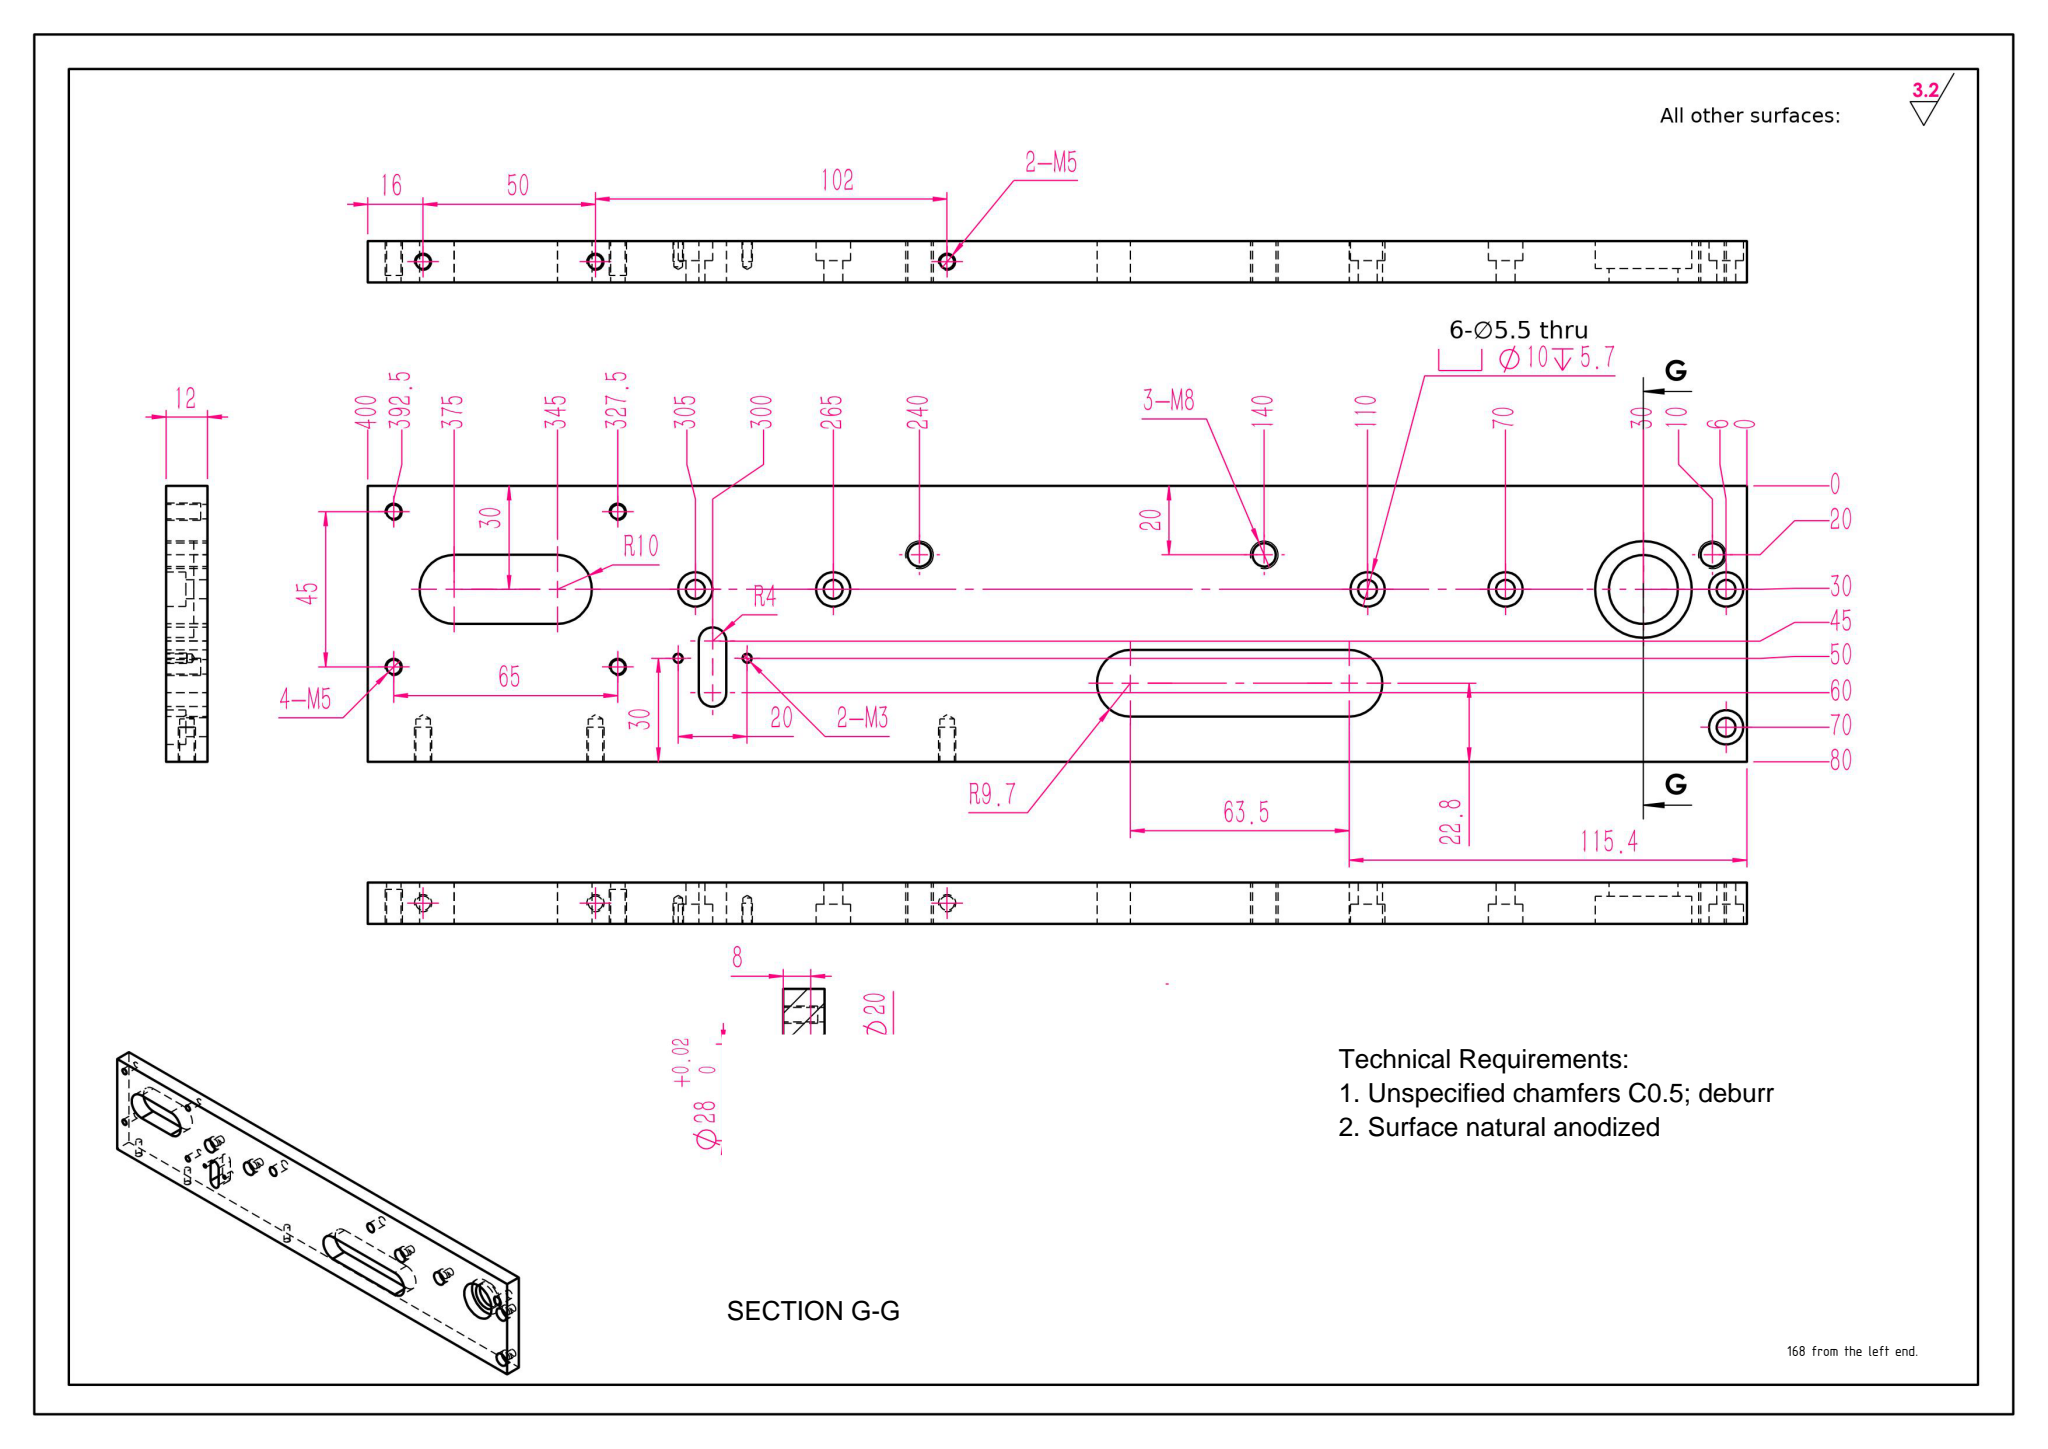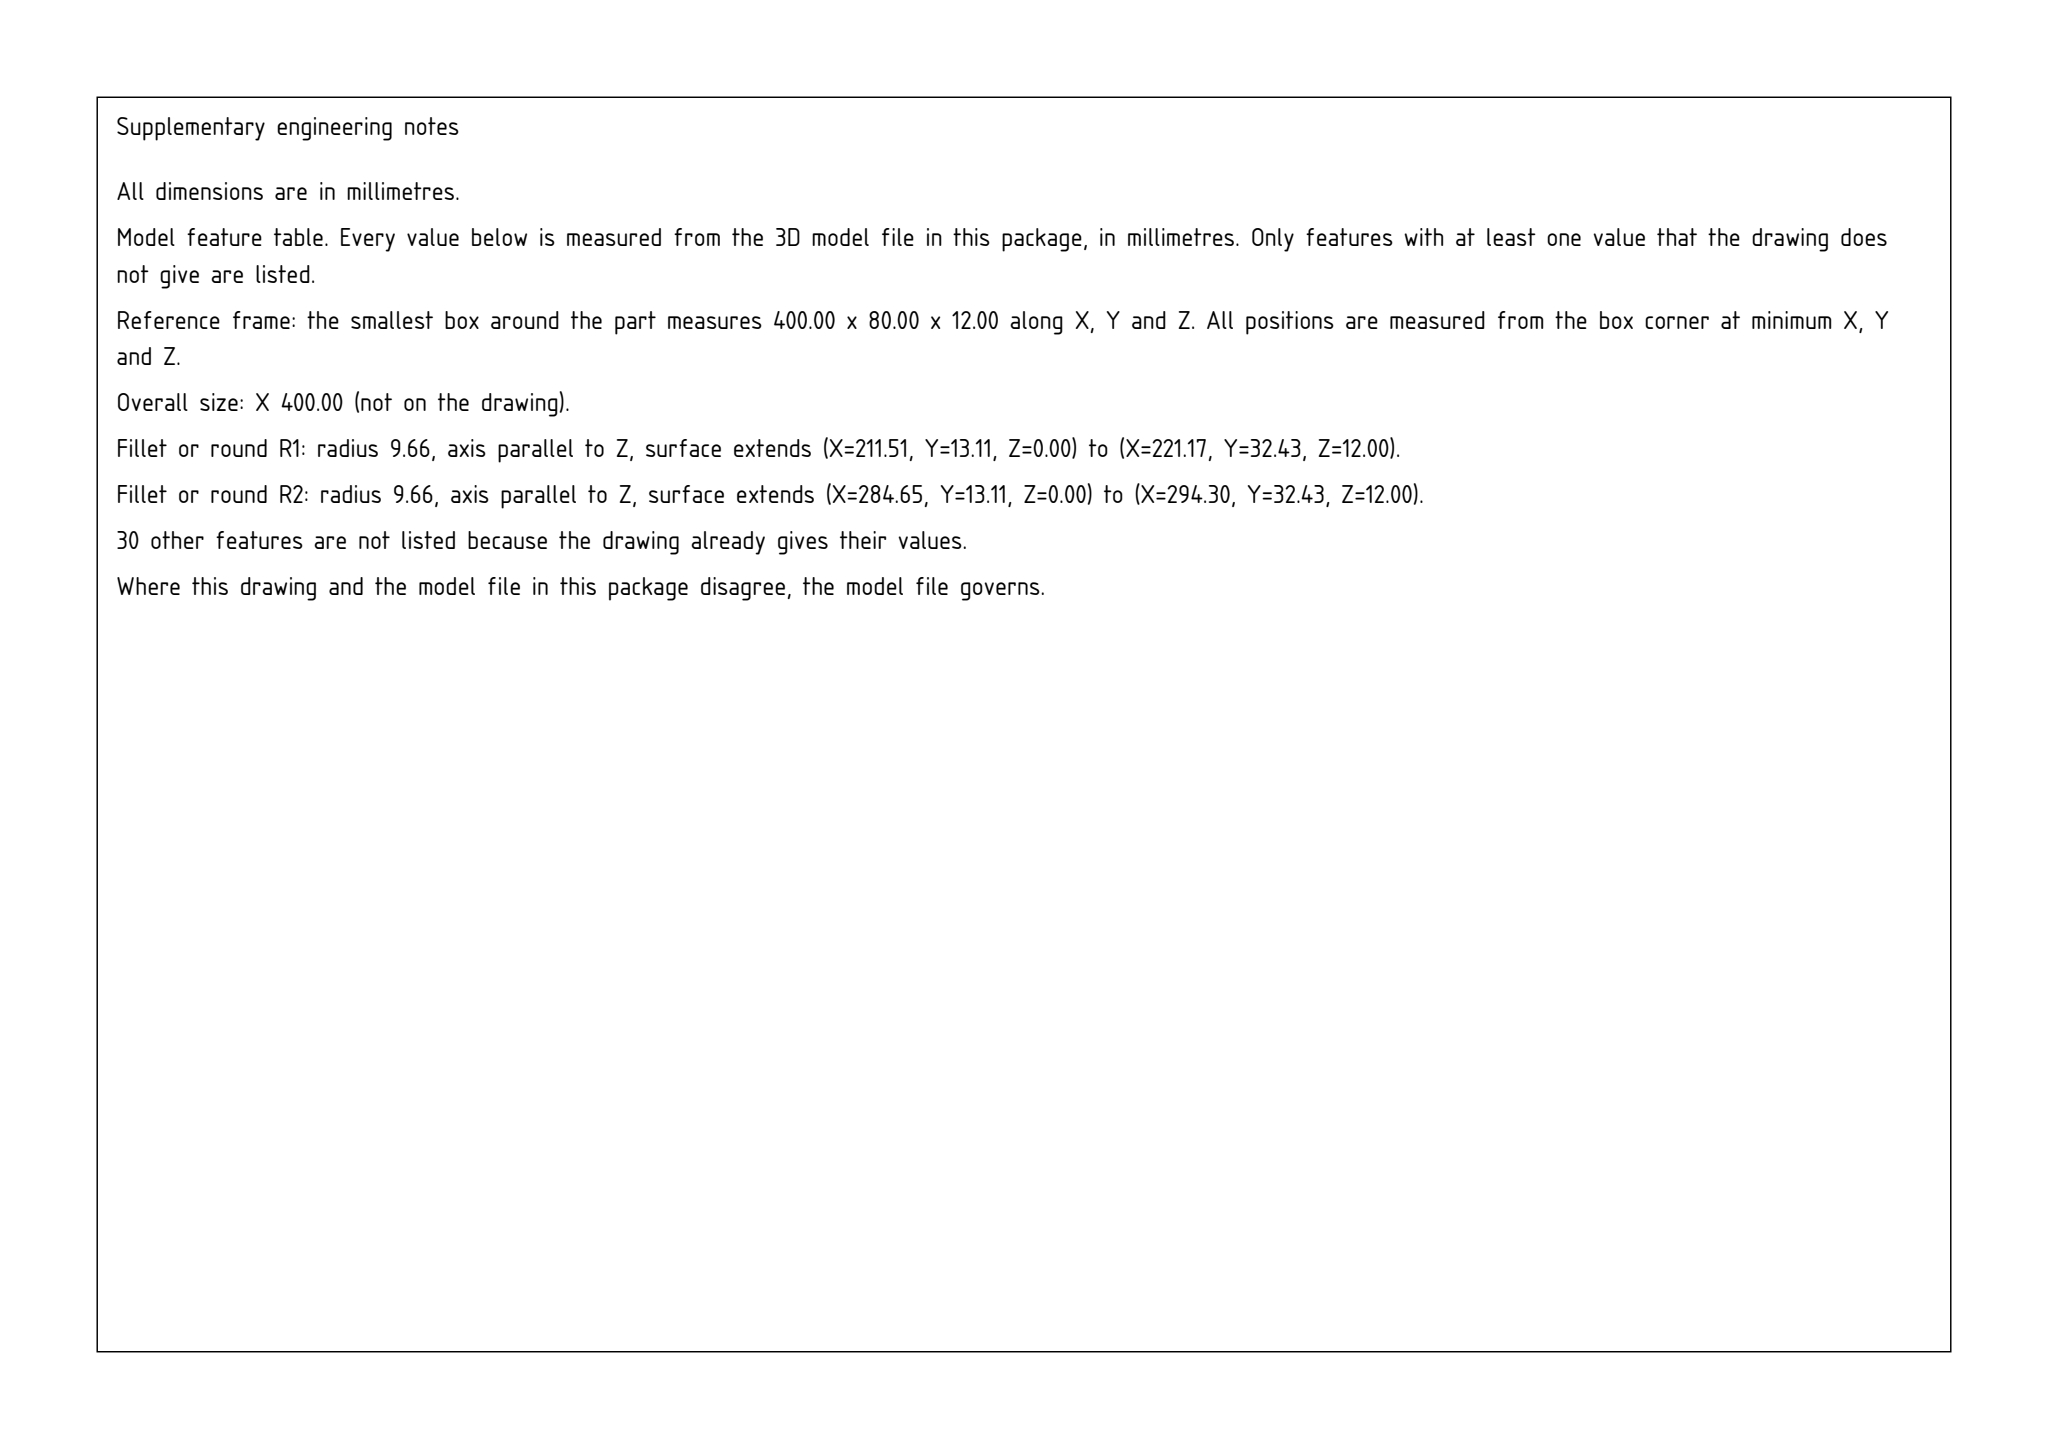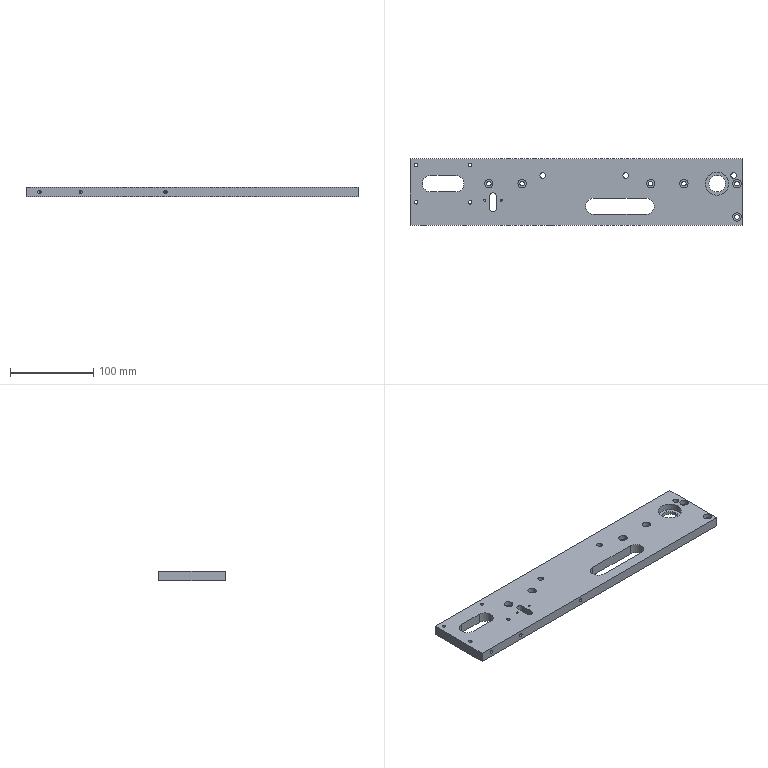Part | SolidWorks | mm | 1 solid | 89 faces | box 400 x 80 x 12 mm | volume 340413 mm3 | cylinder 60 | plane 19 | cone 10 | commonest cylinder face diameters 4.2 x14 10 x12 5.5 x12 6.8 x6 20 x5 2.5 x4 19.312 x3 28 x2
Drawing notes:
2-M3 DP 7.5 FM BACK FACE; DRILL Ø2.5 +118° PT; CL 290 & 310, 50 FM TOP EDGE | from the solid: Ø2.5 z-cyls [90,30] & [110,30] L=7.5 blind, cone 118°; 400-90=310, 400-110=290; 80-30=50
4-M5 THRU pattern (4X Ø4.2 thru, M5 thread): hole centres 7.5 and 52.5 from the top long edge (45 apart) and 7.5 and 72.5 from the left end. | from the solid: cylinders: four Ø4.2 z-axis holes at (7.5,72.5), (72.5,72.5), (7.5,27.5), (72.5,27.5), from z=0 to z=12 (thru 12 thk plate, bbox 400x80x12)
M5 holes in the long edge: Ø4.2 drill 12.4 deep (blind, 118° point), axis at mid-thickness 6.0 from face, entering the y=0 long edge at 16, 66 and 168 from the left end. | from the solid: cylinders: Ø4.2 y-axis holes at x=16, 66, 168, z=6.0, from y=0 to y=12.4; cones 118° ref dia 4.2 at those locations
build123d program:
from build123d import *

# Parameters (mm, degrees)
SKETCH1_W                                            = 400
SKETCH1_H                                            = 80
BOSS_EXTRUDE1_DEPTH                                  = 12
SKETCH2_R                                            = 10
CUT_EXTRUDE1_DEPTH                                   = 205.313
SKETCH3_R                                            = 14
CUT_EXTRUDE2_DEPTH                                   = 8
M5_TAPPED_HOLE1_D                                    = 4.2
M5_TAPPED_HOLE1_DEPTH                                = 12.4
M5_TAPPED_HOLE1_TIP                                  = 1.262
HOLE_SIZE_ACCORDING_TO_HEXAGON_SOCKET_HE_D           = 5.5
HOLE_SIZE_ACCORDING_TO_HEXAGON_SOCKET_HE_CBORE_D     = 10
HOLE_SIZE_ACCORDING_TO_HEXAGON_SOCKET_HE_CBORE_DEPTH = 5.7
M8_TAPPED_HOLE1_D                                    = 6.8
M8_TAPPED_HOLE1_DEPTH                                = 19.75
M8_TAPPED_HOLE1_TIP                                  = 2.043
HOLE_SIZE_ACCORDING_TO_HEXAGON_SOCKE_2_D             = 5.5
HOLE_SIZE_ACCORDING_TO_HEXAGON_SOCKE_2_CBORE_D       = 10
HOLE_SIZE_ACCORDING_TO_HEXAGON_SOCKE_2_CBORE_DEPTH   = 5.7
CUT_EXTRUDE4_DEPTH                                   = 205.313
M3_TAPPED_HOLE1_D                                    = 2.5
M3_TAPPED_HOLE1_DEPTH                                = 7.5
M3_TAPPED_HOLE1_TIP                                  = 0.7511
M5_TAPPED_HOLE2_D                                    = 4.2
M5_TAPPED_HOLE2_DEPTH                                = 12.4
M5_TAPPED_HOLE2_TIP                                  = 1.262
CUT_EXTRUDE5_DEPTH                                   = 57


with BuildPart() as part:
    # Sketch1 → Boss-Extrude1 (new body)
    with BuildSketch(Plane.XY):
        Rectangle(SKETCH1_W, SKETCH1_H)
    extrude(amount=BOSS_EXTRUDE1_DEPTH)

    # Sketch2 → Cut-Extrude1 (cut, through all)
    with BuildSketch(Plane.XY.offset(12)):
        with Locations((170, 10)):
            Circle(SKETCH2_R)
        with BuildLine():
            Line((-175, 20), (-145, 20))
            ThreePointArc((-145, 20), (-135, 10), (-145, 0))
            Line((-145, 0), (-175, 0))
            ThreePointArc((-175, 0), (-185, 10), (-175, 20))
        make_face()
    extrude(amount=-CUT_EXTRUDE1_DEPTH, mode=Mode.SUBTRACT)

    # Sketch3 → Cut-Extrude2 (cut)
    with BuildSketch(Plane.XY.offset(12)):
        with Locations((170, 10)):
            Circle(SKETCH3_R)
    extrude(amount=-CUT_EXTRUDE2_DEPTH, mode=Mode.SUBTRACT)

    # M5 Tapped Hole1
    with Locations(Plane.XY.offset(12)):
        with Locations((-192.5, -12.5), (-127.5, -12.5), (-127.5, 32.5), (-192.5, 32.5)):
            Hole(M5_TAPPED_HOLE1_D / 2, depth=M5_TAPPED_HOLE1_DEPTH)
            with Locations((0, 0, -(M5_TAPPED_HOLE1_DEPTH + M5_TAPPED_HOLE1_TIP / 2))):  # 118° drill point
                Cone(0, M5_TAPPED_HOLE1_D / 2, M5_TAPPED_HOLE1_TIP, mode=Mode.SUBTRACT)

    # Hole Size according to Hexagon Socket He (through all)
    with Locations(Plane.XY.offset(12)):
        with Locations((-105, 10), (-65, 10), (130, 10), (90, 10)):
            CounterBoreHole(HOLE_SIZE_ACCORDING_TO_HEXAGON_SOCKET_HE_D / 2, HOLE_SIZE_ACCORDING_TO_HEXAGON_SOCKET_HE_CBORE_D / 2, HOLE_SIZE_ACCORDING_TO_HEXAGON_SOCKET_HE_CBORE_DEPTH)

    # M8 Tapped Hole1
    with Locations(Plane.XY.offset(12)):
        with Locations((60, 20), (-40, 20), (190, 20)):
            Hole(M8_TAPPED_HOLE1_D / 2, depth=M8_TAPPED_HOLE1_DEPTH)
            with Locations((0, 0, -(M8_TAPPED_HOLE1_DEPTH + M8_TAPPED_HOLE1_TIP / 2))):  # 118° drill point
                Cone(0, M8_TAPPED_HOLE1_D / 2, M8_TAPPED_HOLE1_TIP, mode=Mode.SUBTRACT)

    # Hole Size according to Hexagon Socke 2 (through all)
    with Locations(Plane.XY.offset(12)):
        with Locations((194, -30), (194, 10)):
            CounterBoreHole(HOLE_SIZE_ACCORDING_TO_HEXAGON_SOCKE_2_D / 2, HOLE_SIZE_ACCORDING_TO_HEXAGON_SOCKE_2_CBORE_D / 2, HOLE_SIZE_ACCORDING_TO_HEXAGON_SOCKE_2_CBORE_DEPTH)

    # Sketch15 → Cut-Extrude4 (cut, through all)
    with BuildSketch(Plane.XY.offset(12)):
        with BuildLine():
            Line((-96, -5), (-96, -20))
            ThreePointArc((-96, -20), (-100, -24), (-104, -20))
            Line((-104, -20), (-104, -5))
            ThreePointArc((-104, -5), (-100, -1), (-96, -5))
        make_face()
    extrude(amount=-CUT_EXTRUDE4_DEPTH, mode=Mode.SUBTRACT)

    # M3 Tapped Hole1
    with Locations(Plane.XY.offset(12)):
        with Locations((-110, -10), (-90, -10)):
            Hole(M3_TAPPED_HOLE1_D / 2, depth=M3_TAPPED_HOLE1_DEPTH)
            with Locations((0, 0, -(M3_TAPPED_HOLE1_DEPTH + M3_TAPPED_HOLE1_TIP / 2))):  # 118° drill point
                Cone(0, M3_TAPPED_HOLE1_D / 2, M3_TAPPED_HOLE1_TIP, mode=Mode.SUBTRACT)

    # M5 Tapped Hole2
    with Locations(Plane(origin=(0, -40, 0), x_dir=(-1, 0, 0), z_dir=(0, -1, 0))):
        with Locations((32, -6), (184, -6), (134, -6)):
            Hole(M5_TAPPED_HOLE2_D / 2, depth=M5_TAPPED_HOLE2_DEPTH)
            with Locations((0, 0, -(M5_TAPPED_HOLE2_DEPTH + M5_TAPPED_HOLE2_TIP / 2))):  # 118° drill point
                Cone(0, M5_TAPPED_HOLE2_D / 2, M5_TAPPED_HOLE2_TIP, mode=Mode.SUBTRACT)

    # Sketch21 → Cut-Extrude5 (cut)
    with BuildSketch(Plane(origin=(0, 0, 0), x_dir=(-1, 0, 0), z_dir=(0, 0, -1))):
        with BuildLine():
            Line((-84.649, -7.574), (-21.17, -7.574))
            ThreePointArc((-21.17, -7.574), (-11.514, -17.23), (-21.17, -26.886))
            Line((-21.17, -26.886), (-84.649, -26.886))
            ThreePointArc((-84.649, -26.886), (-94.305, -17.23), (-84.649, -7.574))
        make_face()
    extrude(amount=-CUT_EXTRUDE5_DEPTH, mode=Mode.SUBTRACT)


solid = part.part